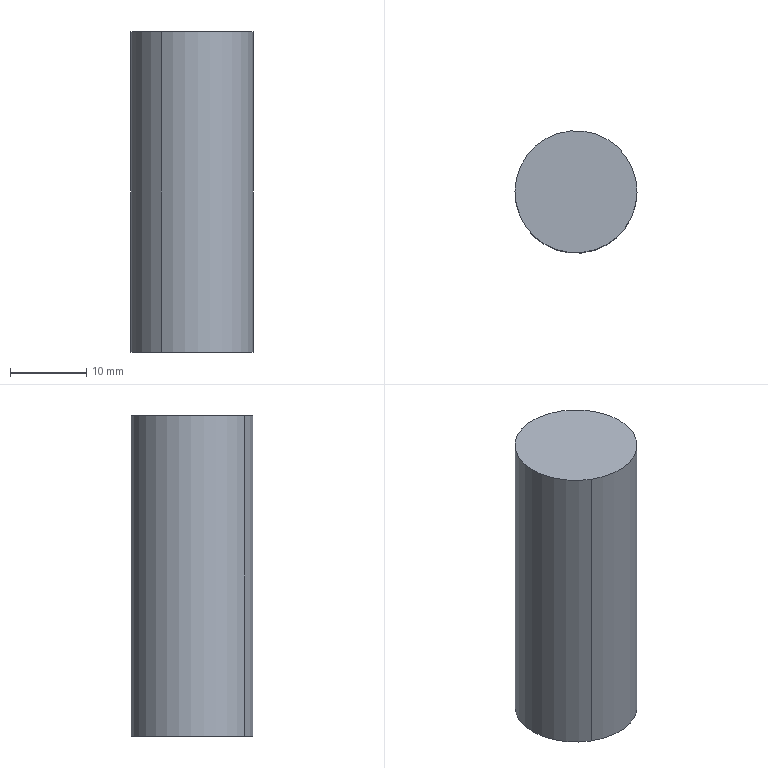Component | SolidWorks | ACQS-32X25PistonRod-2 | 1 solid | 7 faces | box 16 x 16 x 42 mm | volume 7791 mm3 | cylinder 4 | plane 3 | commonest cylinder face diameters 8 x2 16 x2
build123d program:
from build123d import *

# Parameters (mm, degrees)
SKETCH1_R          = 8
EXTRUDE1_DEPTH     = 42
SKETCH6_R          = 4
CUT_EXTRUDE2_DEPTH = 13


with BuildPart() as part:
    # Sketch1 → Extrude1 (new body)
    with BuildSketch(Plane(origin=(0, 0, 0), x_dir=(1, 0, 0), z_dir=(0, 1, 0))):
        with Locations(Location((0, 0, 0), (0, 0, 90))):
            Circle(SKETCH1_R)
    extrude(amount=EXTRUDE1_DEPTH)

    # Sketch6 → Cut-Extrude2 (cut)
    with BuildSketch(Plane(origin=(0, 42, 0), x_dir=(1, 0, 0), z_dir=(0, 1, 0))):
        with Locations(Location((0, 0, 0), (0, 0, 270))):
            Circle(SKETCH6_R)
    extrude(amount=-CUT_EXTRUDE2_DEPTH, mode=Mode.SUBTRACT)


solid = part.part

# Placed as in the assembly
solid = solid.moved(Location((-11.583, 45.872, -35.887), (-90, 0, 0)))
STEP:
#1=COLOUR_RGB('',0.7922,0.8196,0.9333);
#2=FILL_AREA_STYLE_COLOUR('',#1);
#3=FILL_AREA_STYLE('',(#2));
#4=SURFACE_STYLE_FILL_AREA(#3);
#5=SURFACE_SIDE_STYLE('',(#4));
#6=SURFACE_STYLE_USAGE(.BOTH.,#5);
#7=PRESENTATION_STYLE_ASSIGNMENT((#6));
#8=CARTESIAN_POINT('',(-0.376,1.942,-2.555));
#9=VERTEX_POINT('',#8);
#10=CARTESIAN_POINT('',(-0.536,1.67,-2.555));
#11=VERTEX_POINT('',#10);
#12=CARTESIAN_POINT('',(-0.456,1.806,-2.555));
#13=DIRECTION('',(-0.,0.,-1.));
#14=DIRECTION('',(-0.5079,-0.8614,0.));
#15=AXIS2_PLACEMENT_3D('',#12,#13,#14);
#16=CIRCLE('',#15,0.1575);
#17=EDGE_CURVE('',#9,#11,#16,.T.);
#18=ORIENTED_EDGE('',*,*,#17,.F.);
#19=CARTESIAN_POINT('',(-0.376,1.942,-3.066));
#20=VERTEX_POINT('',#19);
#21=CARTESIAN_POINT('',(-0.376,1.942,-2.555));
#22=DIRECTION('',(-0.,0.,-1.));
#23=VECTOR('',#22,39.37);
#24=LINE('',#21,#23);
#25=EDGE_CURVE('',#9,#20,#24,.T.);
#26=ORIENTED_EDGE('',*,*,#25,.T.);
#27=CARTESIAN_POINT('',(-0.536,1.67,-3.066));
#28=VERTEX_POINT('',#27);
#29=CARTESIAN_POINT('',(-0.456,1.806,-3.066));
#30=DIRECTION('',(-0.,0.,-1.));
#31=DIRECTION('',(-0.5079,-0.8614,0.));
#32=AXIS2_PLACEMENT_3D('',#29,#30,#31);
#33=CIRCLE('',#32,0.1575);
#34=EDGE_CURVE('',#20,#28,#33,.T.);
#35=ORIENTED_EDGE('',*,*,#34,.T.);
#36=CARTESIAN_POINT('',(-0.536,1.67,-2.555));
#37=DIRECTION('',(-0.,0.,-1.));
#38=VECTOR('',#37,39.37);
#39=LINE('',#36,#38);
#40=EDGE_CURVE('',#11,#28,#39,.T.);
#41=ORIENTED_EDGE('',*,*,#40,.F.);
#42=EDGE_LOOP('',(#18,#26,#35,#41));
#43=FACE_OUTER_BOUND('',#42,.T.);
#44=CARTESIAN_POINT('',(-0.456,1.806,-2.555));
#45=DIRECTION('',(-0.,0.,-1.));
#46=DIRECTION('',(-0.5079,-0.8614,0.));
#47=AXIS2_PLACEMENT_3D('',#44,#45,#46);
#48=CYLINDRICAL_SURFACE('',#47,0.1575);
#49=ADVANCED_FACE('',(#43),#48,.F.);
#50=CARTESIAN_POINT('',(-0.616,1.535,-3.066));
#51=VERTEX_POINT('',#50);
#52=CARTESIAN_POINT('',(-0.2961,2.077,-3.066));
#53=VERTEX_POINT('',#52);
#54=CARTESIAN_POINT('',(-0.456,1.806,-3.066));
#55=DIRECTION('',(-0.,0.,-1.));
#56=DIRECTION('',(-0.5079,-0.8614,0.));
#57=AXIS2_PLACEMENT_3D('',#54,#55,#56);
#58=CIRCLE('',#57,0.315);
#59=EDGE_CURVE('',#51,#53,#58,.T.);
#60=ORIENTED_EDGE('',*,*,#59,.F.);
#61=CARTESIAN_POINT('',(-0.616,1.535,-1.413));
#62=VERTEX_POINT('',#61);
#63=CARTESIAN_POINT('',(-0.616,1.535,-3.066));
#64=DIRECTION('',(0.,-0.,1.));
#65=VECTOR('',#64,39.37);
#66=LINE('',#63,#65);
#67=EDGE_CURVE('',#51,#62,#66,.T.);
#68=ORIENTED_EDGE('',*,*,#67,.T.);
#69=CARTESIAN_POINT('',(-0.2961,2.077,-1.413));
#70=VERTEX_POINT('',#69);
#71=CARTESIAN_POINT('',(-0.456,1.806,-1.413));
#72=DIRECTION('',(-0.,0.,-1.));
#73=DIRECTION('',(-0.5079,-0.8614,0.));
#74=AXIS2_PLACEMENT_3D('',#71,#72,#73);
#75=CIRCLE('',#74,0.315);
#76=EDGE_CURVE('',#62,#70,#75,.T.);
#77=ORIENTED_EDGE('',*,*,#76,.T.);
#78=CARTESIAN_POINT('',(-0.2961,2.077,-3.066));
#79=DIRECTION('',(0.,-0.,1.));
#80=VECTOR('',#79,39.37);
#81=LINE('',#78,#80);
#82=EDGE_CURVE('',#53,#70,#81,.T.);
#83=ORIENTED_EDGE('',*,*,#82,.F.);
#84=EDGE_LOOP('',(#60,#68,#77,#83));
#85=FACE_OUTER_BOUND('',#84,.T.);
#86=CARTESIAN_POINT('',(-0.456,1.806,-3.066));
#87=DIRECTION('',(0.,-0.,1.));
#88=DIRECTION('',(0.5079,0.8614,0.));
#89=AXIS2_PLACEMENT_3D('',#86,#87,#88);
#90=CYLINDRICAL_SURFACE('',#89,0.315);
#91=ADVANCED_FACE('',(#85),#90,.T.);
#92=ORIENTED_EDGE('',*,*,#67,.F.);
#93=CARTESIAN_POINT('',(-0.456,1.806,-3.066));
#94=DIRECTION('',(-0.,0.,-1.));
#95=DIRECTION('',(-0.5079,-0.8614,0.));
#96=AXIS2_PLACEMENT_3D('',#93,#94,#95);
#97=CIRCLE('',#96,0.315);
#98=EDGE_CURVE('',#53,#51,#97,.T.);
#99=ORIENTED_EDGE('',*,*,#98,.F.);
#100=ORIENTED_EDGE('',*,*,#82,.T.);
#101=CARTESIAN_POINT('',(-0.456,1.806,-1.413));
#102=DIRECTION('',(-0.,0.,-1.));
#103=DIRECTION('',(-0.5079,-0.8614,0.));
#104=AXIS2_PLACEMENT_3D('',#101,#102,#103);
#105=CIRCLE('',#104,0.315);
#106=EDGE_CURVE('',#70,#62,#105,.T.);
#107=ORIENTED_EDGE('',*,*,#106,.T.);
#108=EDGE_LOOP('',(#92,#99,#100,#107));
#109=FACE_OUTER_BOUND('',#108,.T.);
#110=CARTESIAN_POINT('',(-0.456,1.806,-3.066));
#111=DIRECTION('',(0.,-0.,1.));
#112=DIRECTION('',(0.5079,0.8614,0.));
#113=AXIS2_PLACEMENT_3D('',#110,#111,#112);
#114=CYLINDRICAL_SURFACE('',#113,0.315);
#115=ADVANCED_FACE('',(#109),#114,.T.);
#116=CARTESIAN_POINT('',(-0.456,1.806,-3.066));
#117=DIRECTION('',(-0.,0.,-1.));
#118=DIRECTION('',(-0.5079,-0.8614,0.));
#119=AXIS2_PLACEMENT_3D('',#116,#117,#118);
#120=CIRCLE('',#119,0.1575);
#121=EDGE_CURVE('',#28,#20,#120,.T.);
#122=ORIENTED_EDGE('',*,*,#121,.F.);
#123=ORIENTED_EDGE('',*,*,#34,.F.);
#124=EDGE_LOOP('',(#122,#123));
#125=FACE_BOUND('',#124,.T.);
#126=ORIENTED_EDGE('',*,*,#98,.T.);
#127=ORIENTED_EDGE('',*,*,#59,.T.);
#128=EDGE_LOOP('',(#126,#127));
#129=FACE_OUTER_BOUND('',#128,.T.);
#130=CARTESIAN_POINT('',(-0.456,1.806,-3.066));
#131=DIRECTION('',(-0.,0.,-1.));
#132=DIRECTION('',(-0.5079,-0.8614,-0.));
#133=AXIS2_PLACEMENT_3D('',#130,#131,#132);
#134=PLANE('',#133);
#135=ADVANCED_FACE('',(#125,#129),#134,.T.);
#136=ORIENTED_EDGE('',*,*,#106,.F.);
#137=ORIENTED_EDGE('',*,*,#76,.F.);
#138=EDGE_LOOP('',(#136,#137));
#139=FACE_OUTER_BOUND('',#138,.T.);
#140=CARTESIAN_POINT('',(-0.456,1.806,-1.413));
#141=DIRECTION('',(-0.,0.,-1.));
#142=DIRECTION('',(-0.5079,-0.8614,-0.));
#143=AXIS2_PLACEMENT_3D('',#140,#141,#142);
#144=PLANE('',#143);
#145=ADVANCED_FACE('',(#139),#144,.F.);
#146=ORIENTED_EDGE('',*,*,#25,.F.);
#147=CARTESIAN_POINT('',(-0.456,1.806,-2.555));
#148=DIRECTION('',(-0.,0.,-1.));
#149=DIRECTION('',(-0.5079,-0.8614,0.));
#150=AXIS2_PLACEMENT_3D('',#147,#148,#149);
#151=CIRCLE('',#150,0.1575);
#152=EDGE_CURVE('',#11,#9,#151,.T.);
#153=ORIENTED_EDGE('',*,*,#152,.F.);
#154=ORIENTED_EDGE('',*,*,#40,.T.);
#155=ORIENTED_EDGE('',*,*,#121,.T.);
#156=EDGE_LOOP('',(#146,#153,#154,#155));
#157=FACE_OUTER_BOUND('',#156,.T.);
#158=CARTESIAN_POINT('',(-0.456,1.806,-2.555));
#159=DIRECTION('',(-0.,0.,-1.));
#160=DIRECTION('',(-0.5079,-0.8614,0.));
#161=AXIS2_PLACEMENT_3D('',#158,#159,#160);
#162=CYLINDRICAL_SURFACE('',#161,0.1575);
#163=ADVANCED_FACE('',(#157),#162,.F.);
#164=ORIENTED_EDGE('',*,*,#152,.T.);
#165=ORIENTED_EDGE('',*,*,#17,.T.);
#166=EDGE_LOOP('',(#164,#165));
#167=FACE_OUTER_BOUND('',#166,.T.);
#168=CARTESIAN_POINT('',(-0.456,1.806,-2.555));
#169=DIRECTION('',(-0.,0.,-1.));
#170=DIRECTION('',(-0.5079,-0.8614,-0.));
#171=AXIS2_PLACEMENT_3D('',#168,#169,#170);
#172=PLANE('',#171);
#173=ADVANCED_FACE('',(#167),#172,.T.);
#174=CLOSED_SHELL('',(#49,#91,#115,#135,#145,#163,#173));
#175=MANIFOLD_SOLID_BREP('',#174);
#176=STYLED_ITEM('',(#7),#175);
#177=(LENGTH_UNIT()NAMED_UNIT(*)SI_UNIT($,.METRE.));
#178=LENGTH_MEASURE_WITH_UNIT(LENGTH_MEASURE(0.0254),#177);
#179=DIMENSIONAL_EXPONENTS(1.,0.,0.,0.,0.,0.,0.);
#180=(CONVERSION_BASED_UNIT('',#178)LENGTH_UNIT()NAMED_UNIT(#179));
#181=UNCERTAINTY_MEASURE_WITH_UNIT(LENGTH_MEASURE(0.00001),#180,'','');
#182=(NAMED_UNIT(*)PLANE_ANGLE_UNIT()SI_UNIT($,.RADIAN.));
#183=(NAMED_UNIT(*)SI_UNIT($,.STERADIAN.)SOLID_ANGLE_UNIT());
#184=(GEOMETRIC_REPRESENTATION_CONTEXT(3)GLOBAL_UNCERTAINTY_ASSIGNED_CONTEXT((#181))GLOBAL_UNIT_ASSIGNED_CONTEXT((#180,#182,#183))REPRESENTATION_CONTEXT('',''));
#185=MECHANICAL_DESIGN_GEOMETRIC_PRESENTATION_REPRESENTATION('',(#176),#184);
#186=CARTESIAN_POINT('',(0.,0.,0.));
#187=DIRECTION('',(0.,0.,1.));
#188=DIRECTION('',(1.,0.,0.));
#189=AXIS2_PLACEMENT_3D('',#186,#187,#188);
#190=(LENGTH_UNIT()NAMED_UNIT(*)SI_UNIT($,.METRE.));
#191=LENGTH_MEASURE_WITH_UNIT(LENGTH_MEASURE(0.0254),#190);
#192=DIMENSIONAL_EXPONENTS(1.,0.,0.,0.,0.,0.,0.);
#193=(CONVERSION_BASED_UNIT('',#191)LENGTH_UNIT()NAMED_UNIT(#192));
#194=UNCERTAINTY_MEASURE_WITH_UNIT(LENGTH_MEASURE(0.00001),#193,'','');
#195=(NAMED_UNIT(*)PLANE_ANGLE_UNIT()SI_UNIT($,.RADIAN.));
#196=(NAMED_UNIT(*)SI_UNIT($,.STERADIAN.)SOLID_ANGLE_UNIT());
#197=(GEOMETRIC_REPRESENTATION_CONTEXT(3)GLOBAL_UNCERTAINTY_ASSIGNED_CONTEXT((#194))GLOBAL_UNIT_ASSIGNED_CONTEXT((#193,#195,#196))REPRESENTATION_CONTEXT('',''));
#198=ADVANCED_BREP_SHAPE_REPRESENTATION('',(#175,#189),#197);
#199=PRESENTATION_LAYER_ASSIGNMENT('','',(#176));